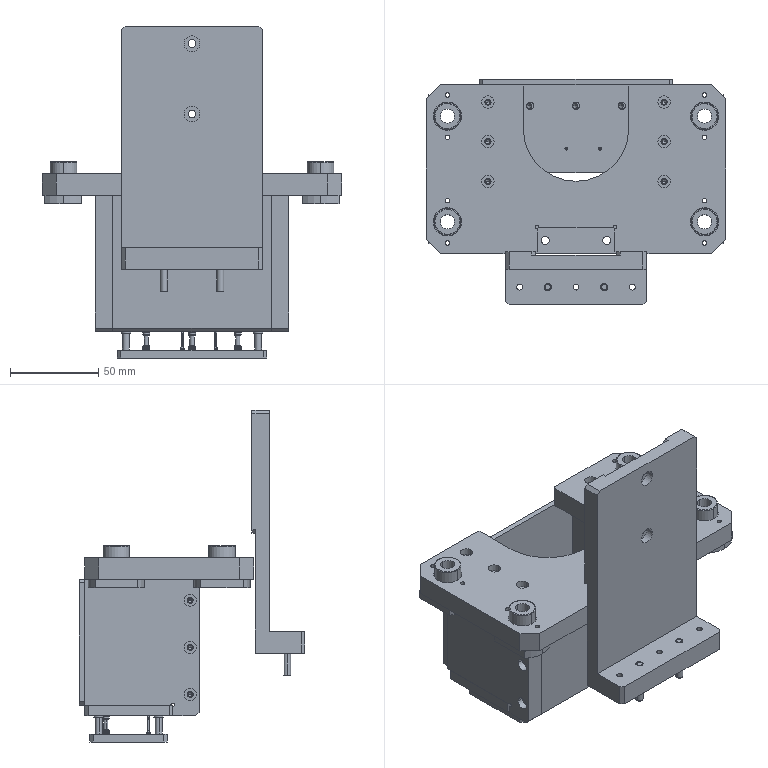Assembly | SolidWorks | mm | 28 component files | 28 solids | 2045 faces | box 170 x 128 x 188.5 mm | volume 512817 mm3 | plane 983 | cylinder 570 | spline 356 | cone 136 | commonest cylinder face diameters 2.5 x96 3.5 x60 7 x52 4 x50 1.57 x30 3.9 x24 5 x20 2.4 x18
Bill of materials:
170423A4-DowelPin4x25 | 2 |  | Solid straight cylindrical pin with chamfered edges at both ends.
170423A4-GKS-100_306_200 | 2 |  | Slender stepped pin with a long upper barrel and a rounded tip, a small collar, a narrower lower shank, and a flared head ending in a serrated, pointed crown.
170423A4-KS-100_30_05 | 2 |  | Long thin-walled tube. One end has part of the wall cut away, leaving a C-shaped section with a step; the other end has a small lip.
170423A4-INGUN_HSS-150_306_400_02_M | 3 |  | Stepped cylindrical shaft: a short plain end section with a small groove, a long main body, a collar, a narrower neck, and an enlarged head with a serrated crown edge.
170423A4-INGUN_KS-150_30_M3_0 | 3 |  | Thin-walled cylindrical tube. One end has a half-cut wall, a small round radial hole sits near that end, and the other end has a thin lip.
170423A4-LME21-d8 | 4 |  | Flanged bushing: a cylindrical boss with a central through bore stands on a flange plate that has two straight parallel sides, two arc-shaped ends, and two through holes.
170423A4-PowerDockingCylinderFixingPlate | 1 |  | L-shaped bracket: an upright plate with two holes on its centerline, and a perpendicular foot with a row of five holes.
170423A4-SafetyPowerProbeFixingPlate1 | 1 |  | Flat rectangular plate with chamfered corners and a symmetric pattern of through holes in several sizes.
170423A4-SafetyPowerProbeFixingPlate2 | 2 |  | Thick rectangular plate/block with three holes along one edge face, three holes through the main face near one side, and a small stepped notch with a relief at one bottom corner.
170423A4-SafetyPowerProbeFixingPlate3 | 1 |  | Rectangular plate with chamfered corners and a large U-shaped cutout open to one long edge, surrounded by many holes.
170423A4-SafetyPowerProbeFixingPlate4 | 1 |  | Plain rectangular block/thick plate with three small holes in a row on one narrow end face.
170423A4-SafetyPowerProbeFixingPlate5 | 1 |  | Thin flat rectangular plate with chamfered corners and four through holes near the corners.
170423A4-SafetyPowerProbeProtectionPlate | 1 |  | Flat rectangular plate with uniform thickness and four chamfered corners. It has a pattern of through holes: four small holes near the corners, three large holes in a row along one long edge, and two medium holes near the opposite long edge.
170423A4-ThimbleSpringGP-2T | 4 |  | Stepped, solid cylindrical pin or shaft. From one end: a short small-diameter stub, a long main body, a thin collar slightly wider than the body, then a shorter lower shank with a smaller diameter than the main body.
Mates:
1. coincident | 170423A4-SafetyPowerProbeFixingPlate1-1 face at (66.593, -20.769, -79.574) dir (0, 0, -1) | 170423A4-GKS100-1/170423A4-KS-100_30_05-1 face at (42.904, 3.532, -79.574) dir (0, 0, 1)
2. concentric | 170423A4-SafetyPowerProbeFixingPlate1-1 face at (42.187, 3.105, -79.574) dir (0, 0, -1) r 0.835 | 170423A4-GKS100-1/170423A4-KS-100_30_05-1 face at (42.187, 3.105, -79.774) dir (0, 0, -1) r 0.835
3. coincident | 170423A4-SafetyPowerProbeFixingPlate1-1 face at (66.593, -20.769, -79.574) dir (0, 0, -1) | 170423A4-GKS100-2/170423A4-KS-100_30_05-1 face at (23.952, 3.532, -79.574) dir (0, 0, 1)
4. concentric | 170423A4-SafetyPowerProbeFixingPlate1-1 face at (23.235, 3.105, -79.574) dir (0, 0, -1) r 0.835 | 170423A4-GKS100-2/170423A4-KS-100_30_05-1 face at (23.235, 3.105, -79.774) dir (0, 0, -1) r 0.835
5. coincident | 170423A4-SafetyPowerProbeFixingPlate1-1 face at (66.593, -20.769, -73.574) dir (0, 0, 1) | 170423A4-SafetyPowerProbeFixingPlate2-1 face at (-26.313, -25.611, -73.574) dir (0, 0, -1)
6. coincident | 170423A4-SafetyPowerProbeFixingPlate1-1 face at (83.687, 39.389, -79.574) dir (0, 1, 0) | 170423A4-SafetyPowerProbeFixingPlate2-1 face at (-26.313, 39.389, -0.07379) dir (0, 1, 0)
7. coincident | 170423A4-SafetyPowerProbeFixingPlate1-1 face at (-26.313, 39.389, -79.574) dir (-1, 0, 0) | 170423A4-SafetyPowerProbeFixingPlate2-1 face at (-26.313, -25.611, -0.07379) dir (-1, 0, 0)
8. coincident | 170423A4-SafetyPowerProbeFixingPlate1-1 face at (66.593, -20.769, -73.574) dir (0, 0, 1) | 170423A4-SafetyPowerProbeFixingPlate2-2 face at (73.687, -25.611, -73.574) dir (0, 0, -1)
9. coincident | 170423A4-SafetyPowerProbeFixingPlate1-1 face at (83.687, 39.389, -79.574) dir (0, 1, 0) | 170423A4-SafetyPowerProbeFixingPlate2-2 face at (73.687, 39.389, -0.07379) dir (0, 1, 0)
10. coincident | 170423A4-SafetyPowerProbeFixingPlate1-1 face at (83.687, 39.389, -79.574) dir (1, 0, 0) | 170423A4-SafetyPowerProbeFixingPlate2-2 face at (83.687, -25.611, -0.07379) dir (1, 0, 0)
11. concentric | 170423A4-ThimbleSpringGP-2T-1 face at (66.187, 31.389, -54.574) dir (0, 0, 1) r 2.5 | 170423A4-SafetyPowerProbeFixingPlate1-1 face at (66.187, 31.389, -79.574) dir (0, 0, -1) r 2.5
12. coincident | 170423A4-SafetyPowerProbeFixingPlate1-1 face at (66.593, -20.769, -79.574) dir (0, 0, -1) | 170423A4-ThimbleSpringGP-2T-1 face at (68.734, 32.424, -79.574) dir (0, 0, 1)
13. coincident | 170423A4-ThimbleSpringGP-2T-2 face at (-8.813, -2.611, -90.074) dir (0, 0, -1) | 170423A4-SafetyPowerProbeProtectionPlate-1 face at (66.593, -20.769, -90.074) dir (0, 0, 1)
14. concentric | 170423A4-ThimbleSpringGP-2T-2 face at (-8.813, -2.611, -54.574) dir (0, 0, 1) r 1.975 | 170423A4-SafetyPowerProbeProtectionPlate-1 face at (-8.813, -2.611, -94.574) dir (0, 0, -1) r 3.5
15. concentric | 170423A4-ThimbleSpringGP-2T-3 face at (-8.813, 31.389, -54.574) dir (0, 0, 1) r 1.975 | 170423A4-SafetyPowerProbeProtectionPlate-1 face at (-8.813, 31.389, -94.574) dir (0, 0, -1) r 3.5
16. coincident | 170423A4-SafetyPowerProbeFixingPlate2-2 face at (73.687, -25.611, -0.07379) dir (0, 0, 1) | 170423A4-SafetyPowerProbeFixingPlate3-1 face at (28.687, -8.611, -0.07379) dir (0, 0, -1)
17. width | 170423A4-SafetyPowerProbeFixingPlate3-1 face at (113.687, -56.611, -2.074) dir (1, 0, 0) | 170423A4-SafetyPowerProbeFixingPlate3-1 face at (-56.313, -56.611, -2.074) dir (-1, 0, 0) | 170423A4-SafetyPowerProbeFixingPlate2-1 face at (-26.313, -25.611, -0.07379) dir (-1, 0, 0) | 170423A4-SafetyPowerProbeFixingPlate2-2 face at (83.687, -25.611, -0.07379) dir (1, 0, 0)
18. coincident | 170423A4-SafetyPowerProbeFixingPlate2-2 face at (73.687, 39.389, -0.07379) dir (0, 1, 0) | 170423A4-SafetyPowerProbeFixingPlate3-1 face at (-56.313, 39.389, -2.074) dir (0, 1, 0)
19. coincident | 170423A4-SafetyPowerProbeFixingPlate3-1 face at (28.687, -8.611, -2.074) dir (0, 0, -1) | 170423A4-LME21-d8-1 face at (-44.313, -38.611, -2.074) dir (0, 0, 1)
20. concentric | 170423A4-SafetyPowerProbeFixingPlate3-1 face at (-44.313, -38.611, 9.926) dir (0, 0, -1) r 8 | 170423A4-LME21-d8-1 face at (-44.313, -38.611, -7.074) dir (0, 0, 1) r 7.5
21. parallel | 170423A4-SafetyPowerProbeFixingPlate3-1 face at (-56.313, -56.611, -2.074) dir (-1, 0, 0) | 170423A4-LME21-d8-1 face at (-54.813, -26.538, -2.074) dir (-1, 0, 0)
22. concentric | 170423A4-SafetyPowerProbeFixingPlate3-1 face at (-44.313, 21.389, 9.926) dir (0, 0, -1) r 8 | 170423A4-LME21-d8-2 face at (-44.313, 21.389, -7.074) dir (0, 0, 1) r 7.5
23. coincident | 170423A4-SafetyPowerProbeFixingPlate3-1 face at (28.687, -8.611, -2.074) dir (0, 0, -1) | 170423A4-LME21-d8-2 face at (-44.313, 21.389, -2.074) dir (0, 0, 1)
24. parallel | 170423A4-SafetyPowerProbeFixingPlate3-1 face at (-56.313, -56.611, -2.074) dir (-1, 0, 0) | 170423A4-LME21-d8-2 face at (-54.813, 33.462, -2.074) dir (-1, 0, 0)
25. coincident | 170423A4-SafetyPowerProbeFixingPlate3-1 face at (28.687, -8.611, -2.074) dir (0, 0, -1) | 170423A4-LME21-d8-3 face at (101.687, -38.611, -2.074) dir (0, 0, 1)
26. concentric | 170423A4-SafetyPowerProbeFixingPlate3-1 face at (101.687, -38.611, 9.926) dir (0, 0, -1) r 8 | 170423A4-LME21-d8-3 face at (101.687, -38.611, -7.074) dir (0, 0, 1) r 7.5
27. parallel | 170423A4-SafetyPowerProbeFixingPlate3-1 face at (113.687, -56.611, -2.074) dir (1, 0, 0) | 170423A4-LME21-d8-3 face at (112.187, -50.684, -2.074) dir (1, 0, 0)
28. coincident | 170423A4-SafetyPowerProbeFixingPlate3-1 face at (28.687, -8.611, -2.074) dir (0, 0, -1) | 170423A4-LME21-d8-4 face at (101.687, 21.389, -2.074) dir (0, 0, 1)
29. concentric | 170423A4-SafetyPowerProbeFixingPlate3-1 face at (101.687, 21.389, 9.926) dir (0, 0, -1) r 8 | 170423A4-LME21-d8-4 face at (101.687, 21.389, -7.074) dir (0, 0, 1) r 7.5
30. parallel | 170423A4-SafetyPowerProbeFixingPlate3-1 face at (113.687, -56.611, -2.074) dir (1, 0, 0) | 170423A4-LME21-d8-4 face at (112.187, 9.316, -2.074) dir (1, 0, 0)
31. coincident | 170423A4-SafetyPowerProbeFixingPlate2-2 face at (73.687, -25.611, -0.07379) dir (0, -1, 0) | 170423A4-SafetyPowerProbeFixingPlate4-1 face at (28.687, -25.611, -40.824) dir (0, -1, 0)
32. coincident | 170423A4-SafetyPowerProbeFixingPlate2-2 face at (73.687, -25.611, -0.07379) dir (-1, 0, 0) | 170423A4-SafetyPowerProbeFixingPlate4-1 face at (73.687, -25.611, -79.574) dir (1, 0, 0)
33. coincident | 170423A4-SafetyPowerProbeFixingPlate2-2 face at (83.687, -25.611, -79.574) dir (0, 0, -1) | 170423A4-SafetyPowerProbeFixingPlate4-1 face at (73.687, -25.611, -79.574) dir (0, 0, -1)
34. coincident | 170423A4-SafetyPowerProbeFixingPlate1-1 face at (83.687, 39.389, -79.574) dir (0, 1, 0) | 170423A4-SafetyPowerProbeFixingPlate5-1 face at (28.687, 39.389, -37.824) dir (0, -1, 0)
35. width | 170423A4-SafetyPowerProbeFixingPlate1-1 face at (83.687, 39.389, -79.574) dir (1, 0, 0) | 170423A4-SafetyPowerProbeFixingPlate1-1 face at (-26.313, 39.389, -79.574) dir (-1, 0, 0) | 170423A4-SafetyPowerProbeFixingPlate5-1 face at (-26.313, 42.389, -2.074) dir (-1, 0, 0) | 170423A4-SafetyPowerProbeFixingPlate5-1 face at (83.687, 42.389, -2.074) dir (1, 0, 0)
36. coincident | 170423A4-SafetyPowerProbeFixingPlate1-1 face at (66.593, -20.769, -79.574) dir (0, 0, -1) | 170423A4-INGUN HSS150-1/170423A4-INGUN_KS-150_30_M3_0-1 face at (56.687, 27.389, -79.574) dir (0, 0, 1)
37. concentric | 170423A4-SafetyPowerProbeFixingPlate1-1 face at (54.687, 27.389, -79.574) dir (0, 0, -1) r 2 | 170423A4-INGUN HSS150-1/170423A4-INGUN_KS-150_30_M3_0-1 face at (54.687, 27.389, -63.525) dir (0, 0, 1) r 2
38. coincident | 170423A4-SafetyPowerProbeFixingPlate1-1 face at (66.593, -20.769, -79.574) dir (0, 0, -1) | 170423A4-INGUN HSS150-2/170423A4-INGUN_KS-150_30_M3_0-1 face at (30.687, 27.389, -79.574) dir (0, 0, 1)
39. concentric | 170423A4-SafetyPowerProbeFixingPlate1-1 face at (28.687, 27.389, -79.574) dir (0, 0, -1) r 2 | 170423A4-INGUN HSS150-2/170423A4-INGUN_KS-150_30_M3_0-1 face at (28.687, 27.389, -63.525) dir (0, 0, 1) r 2
40. coincident | 170423A4-SafetyPowerProbeFixingPlate1-1 face at (66.593, -20.769, -79.574) dir (0, 0, -1) | 170423A4-INGUN HSS150-3/170423A4-INGUN_KS-150_30_M3_0-1 face at (4.687, 27.389, -79.574) dir (0, 0, 1)
41. concentric | 170423A4-SafetyPowerProbeFixingPlate1-1 face at (2.687, 27.389, -79.574) dir (0, 0, -1) r 2 | 170423A4-INGUN HSS150-3/170423A4-INGUN_KS-150_30_M3_0-1 face at (2.687, 27.389, -63.525) dir (0, 0, 1) r 2
42. coincident | 170423A4-SafetyPowerProbeFixingPlate3-1 face at (28.687, -8.611, -2.074) dir (0, 0, -1) | 170423A4-SafetyPowerProbeFixingPlate5-1 face at (83.687, 42.389, -2.074) dir (0, 0, 1)
43. concentric | 170423A4-PowerDockingCylinderFixingPlate-1 face at (44.687, -75.611, -44.074) dir (0, 0, -1) r 2 | 170423A4-DowelPin4x25-1 face at (44.687, -75.611, -32.074) dir (0, 0, -1) r 2
44. coincident | 170423A4-PowerDockingCylinderFixingPlate-1 face at (68.687, -85.611, -32.074) dir (0, 0, 1) | 170423A4-DowelPin4x25-1 face at (44.687, -75.611, -32.074) dir (0, 0, 1)
45. concentric | 170423A4-PowerDockingCylinderFixingPlate-1 face at (12.687, -75.611, -44.074) dir (0, 0, -1) r 2 | 170423A4-DowelPin4x25-2 face at (12.687, -75.611, -32.074) dir (0, 0, -1) r 2
46. coincident | 170423A4-PowerDockingCylinderFixingPlate-1 face at (68.687, -85.611, -32.074) dir (0, 0, 1) | 170423A4-DowelPin4x25-2 face at (12.687, -75.611, -32.074) dir (0, 0, 1)
47. concentric | 170423A4-GKS-100_306_200-1 face at (3.933, 1.415, 26.028) dir (0, -1, 0) r 0.683 | 170423A4-KS-100_30_05-1 face at (3.933, 24.595, 26.028) dir (0, 1, 0) r 0.835
48. distance | 170423A4-GKS-100_306_200-1 vertex at (3.094, 34.895, 26.471) dir (1, 0, 0) | 170423A4-KS-100_30_05-1 face at (4.759, 24.395, 26.148) dir (0, -1, 0)
49. concentric | 170423A4-INGUN_KS-150_30_M3_0-1 face at (1.167, 23.855, 43.46) dir (0, -1, 0) r 2 | 170423A4-INGUN_HSS-150_306_400_02_M-1 face at (1.167, 43.316, 43.46) dir (0, 1, 0) r 1.75
50. coincident | 170423A4-INGUN_KS-150_30_M3_0-1 face at (3.317, 40.204, 43.46) dir (0, 1, 0) | 170423A4-INGUN_HSS-150_306_400_02_M-1 face at (1.89, 40.204, 41.866) dir (0, -1, 0)